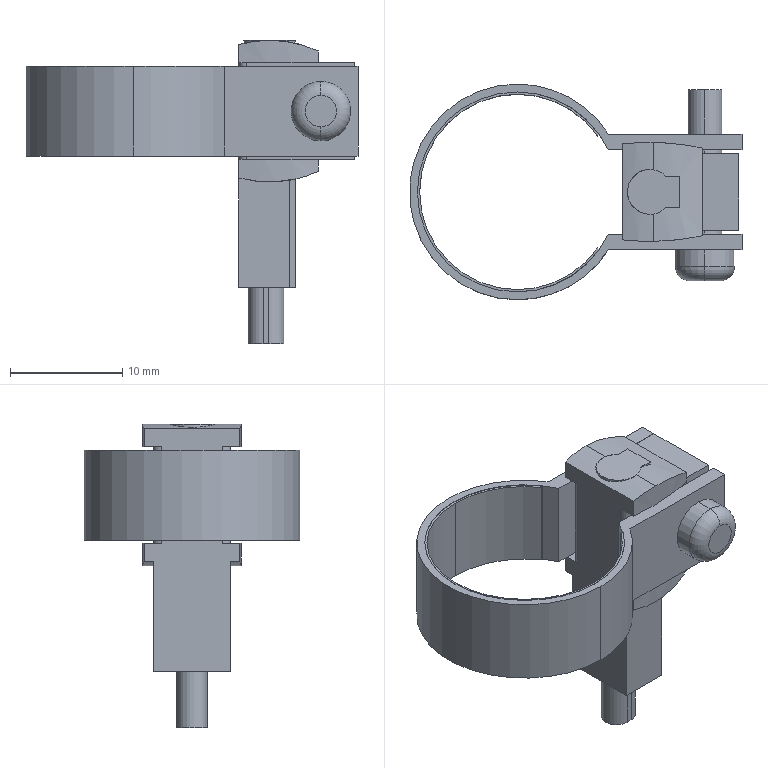Component | SolidWorks | F-YBCDJ2RKA16-125-M9NL(0_0_0)-1_F-YBCJ2_D-M9N_BJ2-016_BJ3-1(16_125_18_3)-2 | 1 solid | 90 faces | volume 1810 mm3 | plane 49 | cylinder 39 | torus 2 | commonest cylinder face diameters 3 x6 4 x6 44 x6 20.776 x5 17.8 x4 17.4 x3 19.2 x3 5.302 x2